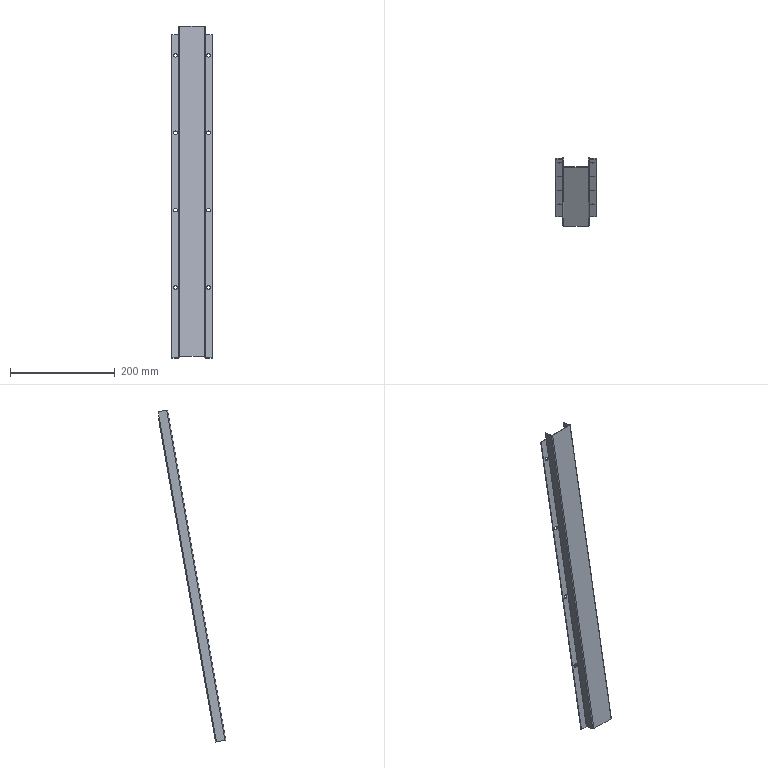Component | SolidWorks | Assembly2-1_WaterproofSlot2-2 | 1 solid | 55 faces | volume 106813 mm3 | plane 31 | cylinder 24 | commonest cylinder face diameters 7 x16 3.4 x4 0.4 x4